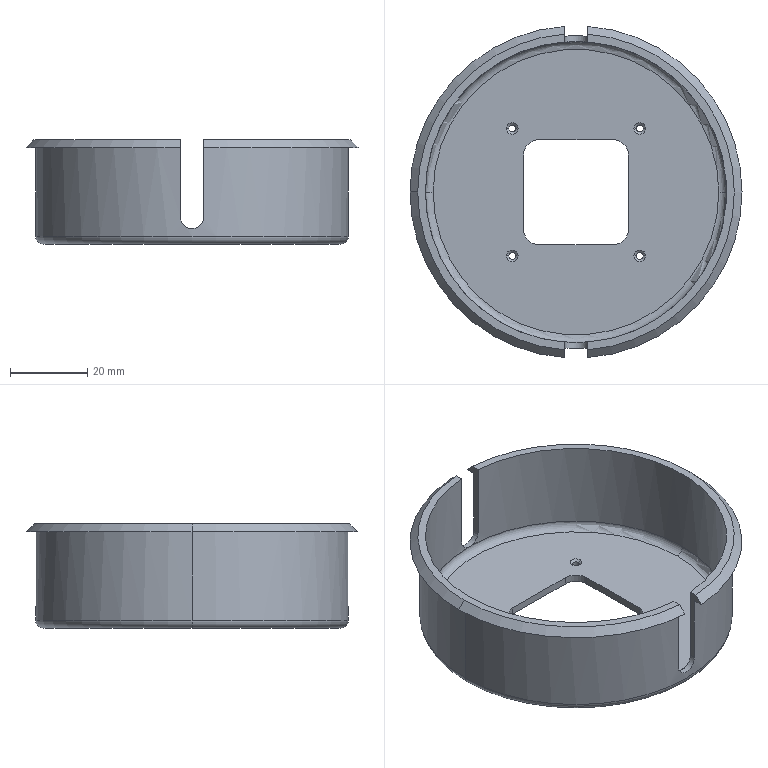Component | SolidWorks | GMotorCover-2 | 1 solid | 48 faces | volume 18528 mm3 | cylinder 19 | plane 14 | cone 11 | torus 4 | commonest cylinder face diameters 1.778 x8 8 x4 78 x3 81 x2 6 x2